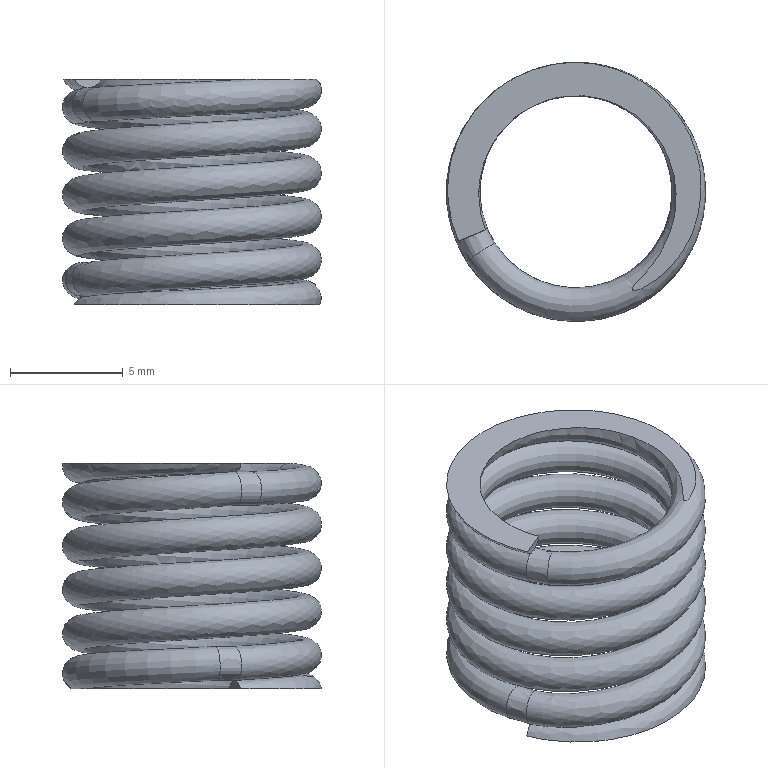Component | NX | SPRING_CYLINDER_COMPRESSION_1 | 1 solid | 9 faces | volume 301 mm3 | spline 5 | plane 4